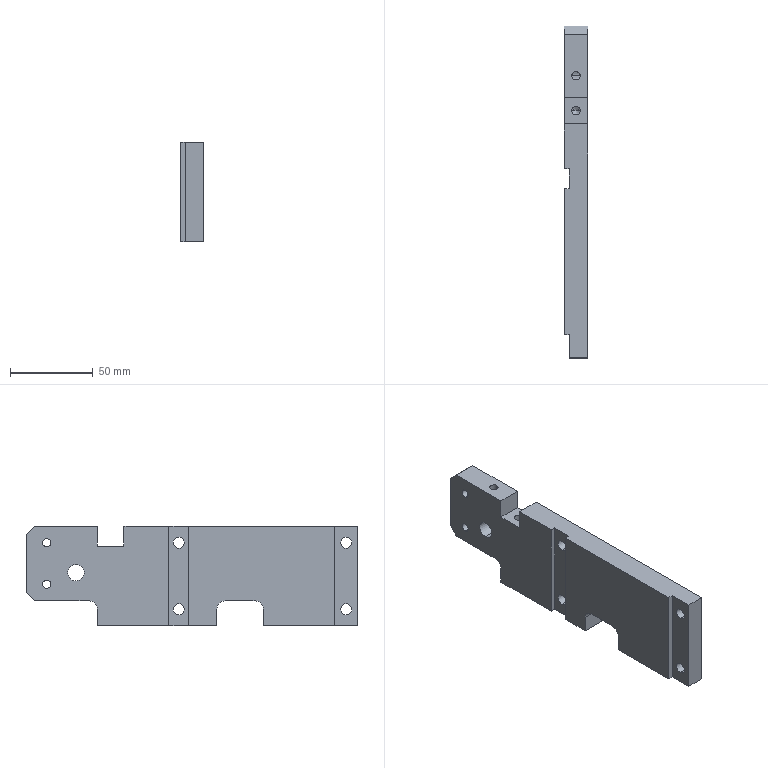Component | SolidWorks | OPW-05-001-1 | 1 solid | 75 faces | box 14 x 200 x 60 mm | volume 138889 mm3 | cylinder 37 | plane 28 | cone 10 | commonest cylinder face diameters 5 x16 11 x8 6.6 x8 10 x5
build123d program:
from build123d import *

# Parameters (mm, degrees)
SKETCH1_W                                       = 60
SKETCH1_H                                       = 200
BOSS_EXTRUDE1_DEPTH                             = 7
SKETCH2_W                                       = 60
SKETCH2_H                                       = 14
SKETCH2_H_2                                     = 12
CUT_EXTRUDE1_DEPTH                              = 3
M6_HEX_SOCKET_HEAD_CAP_SCREW_CBORE1_D           = 6.6
M6_HEX_SOCKET_HEAD_CAP_SCREW_CBORE1_CBORE_D     = 11
M6_HEX_SOCKET_HEAD_CAP_SCREW_CBORE1_CBORE_DEPTH = 6
M6_TAPPED_HOLE1_D                               = 5
M6_TAPPED_HOLE1_DEPTH                           = 17
M6_TAPPED_HOLE1_TIP                             = 1.502
CUT_EXTRUDE2_REACH                              = 107.338
SKETCH7_W                                       = 15
SKETCH7_H                                       = 28
SKETCH7_H_2                                     = 43
FILLET1_R                                       = 5
CUT_EXTRUDE3_REACH                              = 107.338
SKETCH8_R                                       = 5
M6_TAPPED_HOLE2_REACH                           = 118.829
M6_TAPPED_HOLE2_BORE_R                          = 2.5
CHAMFER1_SIZE                                   = 5
CUT_EXTRUDE4_REACH                              = 107.338
SKETCH11_W                                      = 12
SKETCH11_H                                      = 16
M6_TAPPED_HOLE3_D                               = 5
M6_TAPPED_HOLE3_DEPTH                           = 17
M6_TAPPED_HOLE3_TIP                             = 1.502
M6_TAPPED_HOLE4_D                               = 5
M6_TAPPED_HOLE5_D                               = 5
M6_TAPPED_HOLE5_DEPTH                           = 15
M6_TAPPED_HOLE5_TIP                             = 1.502


with BuildPart() as part:
    # Sketch1 → Boss-Extrude1 (new, symmetric)
    with BuildSketch(Plane.XY):
        Rectangle(SKETCH1_W, SKETCH1_H)
    extrude(amount=BOSS_EXTRUDE1_DEPTH, both=True)

    # Sketch2 → Cut-Extrude1 (cut)
    with BuildSketch(Plane(origin=(0, 0, 7), x_dir=(-1, 0, 0), z_dir=(0, 0, -1))):
        with Locations((0, -93)):
            Rectangle(SKETCH2_W, SKETCH2_H)
        with Locations((0, 8)):
            Rectangle(SKETCH2_W, SKETCH2_H_2)
    extrude(amount=CUT_EXTRUDE1_DEPTH, mode=Mode.SUBTRACT)

    # M6 Hex Socket Head Cap Screw CBORE1 (through all)
    with Locations(Plane(origin=(-4.619, -16.722, -7), x_dir=(1, 0, 0), z_dir=(0, 0, -1))):
        with Locations((-15.381, 76.278), (24.619, 76.278), (24.619, -24.722), (-15.381, -24.722)):
            CounterBoreHole(M6_HEX_SOCKET_HEAD_CAP_SCREW_CBORE1_D / 2, M6_HEX_SOCKET_HEAD_CAP_SCREW_CBORE1_CBORE_D / 2, M6_HEX_SOCKET_HEAD_CAP_SCREW_CBORE1_CBORE_DEPTH)

    # M6 Tapped Hole1
    with Locations(Plane(origin=(-30, 130, 7), x_dir=(0, 0, 1), z_dir=(-1, 0, 0))):
        with Locations((-7, -181), (-7, -199)):
            Hole(M6_TAPPED_HOLE1_D / 2, depth=M6_TAPPED_HOLE1_DEPTH)
            with Locations((0, 0, -(M6_TAPPED_HOLE1_DEPTH + M6_TAPPED_HOLE1_TIP / 2))):  # 118° drill point
                Cone(0, M6_TAPPED_HOLE1_D / 2, M6_TAPPED_HOLE1_TIP, mode=Mode.SUBTRACT)

    # Sketch7 → Cut-Extrude2 (cut, up to next)
    with BuildSketch(Plane.XY.offset(7), mode=Mode.PRIVATE) as cut_extrude2_sk1:
        with Locations((-22.5, -29)):
            Rectangle(SKETCH7_W, SKETCH7_H)
    cut_extrude2_tool1 = extrude(cut_extrude2_sk1.sketch, amount=-CUT_EXTRUDE2_REACH, mode=Mode.PRIVATE) & part.part
    # Sketch7 → Cut-Extrude2 (cut, up to next)
    with BuildSketch(Plane.XY.offset(7), mode=Mode.PRIVATE) as cut_extrude2_sk2:
        with Locations((-22.5, 78.5)):
            Rectangle(SKETCH7_W, SKETCH7_H_2)
    cut_extrude2_tool2 = extrude(cut_extrude2_sk2.sketch, amount=-CUT_EXTRUDE2_REACH, mode=Mode.PRIVATE) & part.part
    add(cut_extrude2_tool1.solids().sort_by_distance((-22.5, -29, 7))[0], mode=Mode.SUBTRACT)
    add(cut_extrude2_tool2.solids().sort_by_distance((-22.5, 78.5, 7))[0], mode=Mode.SUBTRACT)

    # Fillet1
    fillet1_edges = [part.edges().sort_by_distance(p)[0] for p in [
        (-15, 57, 0),
        (-15, -15, 0),
        (-15, -43, 0),
    ]]
    fillet(fillet1_edges, radius=FILLET1_R)

    # Sketch8 → Cut-Extrude3 (cut, up to next)
    with BuildSketch(Plane(origin=(0, 0, -7), x_dir=(-1, 0, 0), z_dir=(0, 0, -1)), mode=Mode.PRIVATE) as cut_extrude3_sk1:
        with Locations((-2, 70)):
            Circle(SKETCH8_R)
    cut_extrude3_tool1 = extrude(cut_extrude3_sk1.sketch, amount=-CUT_EXTRUDE3_REACH, mode=Mode.PRIVATE) & part.part
    add(cut_extrude3_tool1.solids().sort_by_distance((2, 70, -7))[0], mode=Mode.SUBTRACT)

    # M6 Tapped Hole2 bore → M6 Tapped Hole2 (cut, up to next)
    with BuildSketch(Plane(origin=(30, 0, 0), x_dir=(0, 0, -1), z_dir=(1, 0, 0)), mode=Mode.PRIVATE) as m6_tapped_hole2_sk1:
        with Locations((0, 70)):
            Circle(M6_TAPPED_HOLE2_BORE_R)
    m6_tapped_hole2_tool1 = extrude(m6_tapped_hole2_sk1.sketch, amount=-M6_TAPPED_HOLE2_REACH, mode=Mode.PRIVATE) & part.part
    add(m6_tapped_hole2_tool1.solids().sort_by_distance((30, 70, 0))[0], mode=Mode.SUBTRACT)

    # Chamfer1
    chamfer1_edges = [part.edges().sort_by_distance(p)[0] for p in [
        (-15, 100, 0),
        (30, 100, 0),
    ]]
    chamfer(chamfer1_edges, length=CHAMFER1_SIZE)

    # Sketch11 → Cut-Extrude4 (cut, up to next)
    with BuildSketch(Plane(origin=(0, 0, -7), x_dir=(-1, 0, 0), z_dir=(0, 0, -1)), mode=Mode.PRIVATE) as cut_extrude4_sk1:
        with Locations((-24, 49)):
            Rectangle(SKETCH11_W, SKETCH11_H)
    cut_extrude4_tool1 = extrude(cut_extrude4_sk1.sketch, amount=-CUT_EXTRUDE4_REACH, mode=Mode.PRIVATE) & part.part
    add(cut_extrude4_tool1.solids().sort_by_distance((24, 49, -7))[0], mode=Mode.SUBTRACT)

    # M6 Tapped Hole3
    with Locations(Plane(origin=(18, 0, 0), x_dir=(0, 0, -1), z_dir=(1, 0, 0))):
        with Locations((0, 49)):
            Hole(M6_TAPPED_HOLE3_D / 2, depth=M6_TAPPED_HOLE3_DEPTH)
            with Locations((0, 0, -(M6_TAPPED_HOLE3_DEPTH + M6_TAPPED_HOLE3_TIP / 2))):  # 118° drill point
                Cone(0, M6_TAPPED_HOLE3_D / 2, M6_TAPPED_HOLE3_TIP, mode=Mode.SUBTRACT)

    # M6 Tapped Hole4 (through all)
    with Locations(Plane(origin=(0, 0, -7), x_dir=(-1, 0, 0), z_dir=(0, 0, -1))):
        with Locations((-20, 87.5), (5, 87.5)):
            Hole(M6_TAPPED_HOLE4_D / 2)

    # M6 Tapped Hole5
    with Locations(Plane.ZY.offset(30)):
        with Locations((0, 0), (0, 45)):
            Hole(M6_TAPPED_HOLE5_D / 2, depth=M6_TAPPED_HOLE5_DEPTH)
            with Locations((0, 0, -(M6_TAPPED_HOLE5_DEPTH + M6_TAPPED_HOLE5_TIP / 2))):  # 118° drill point
                Cone(0, M6_TAPPED_HOLE5_D / 2, M6_TAPPED_HOLE5_TIP, mode=Mode.SUBTRACT)


solid = part.part

# Placed as in the assembly
solid = solid.moved(Location((38.096, 141.999, 0), (0, -90, 0)))